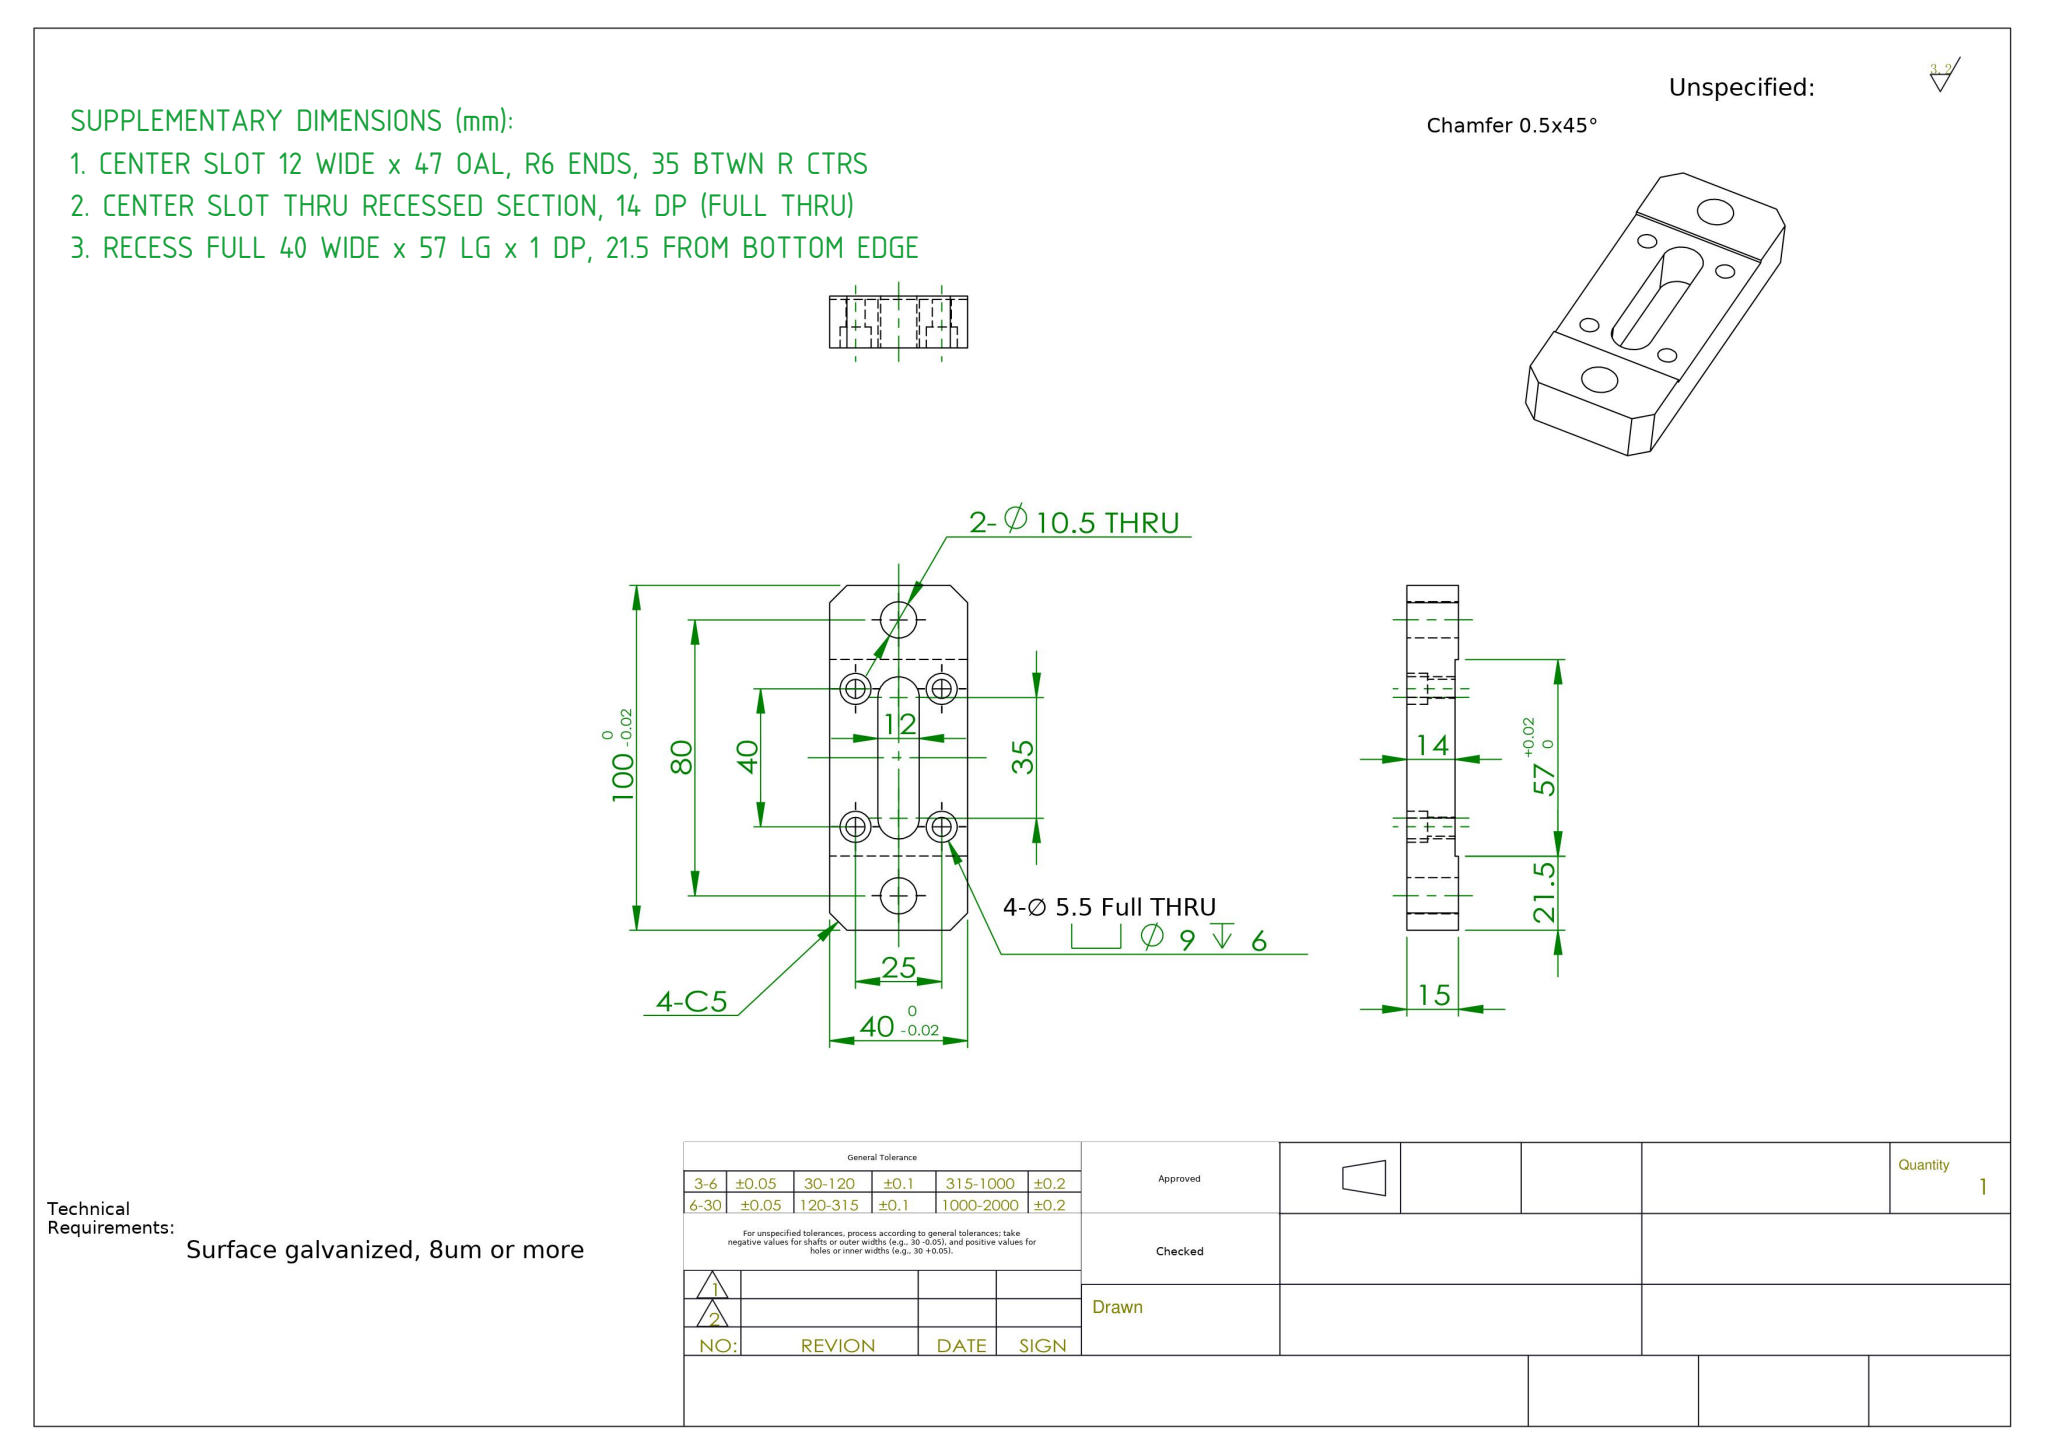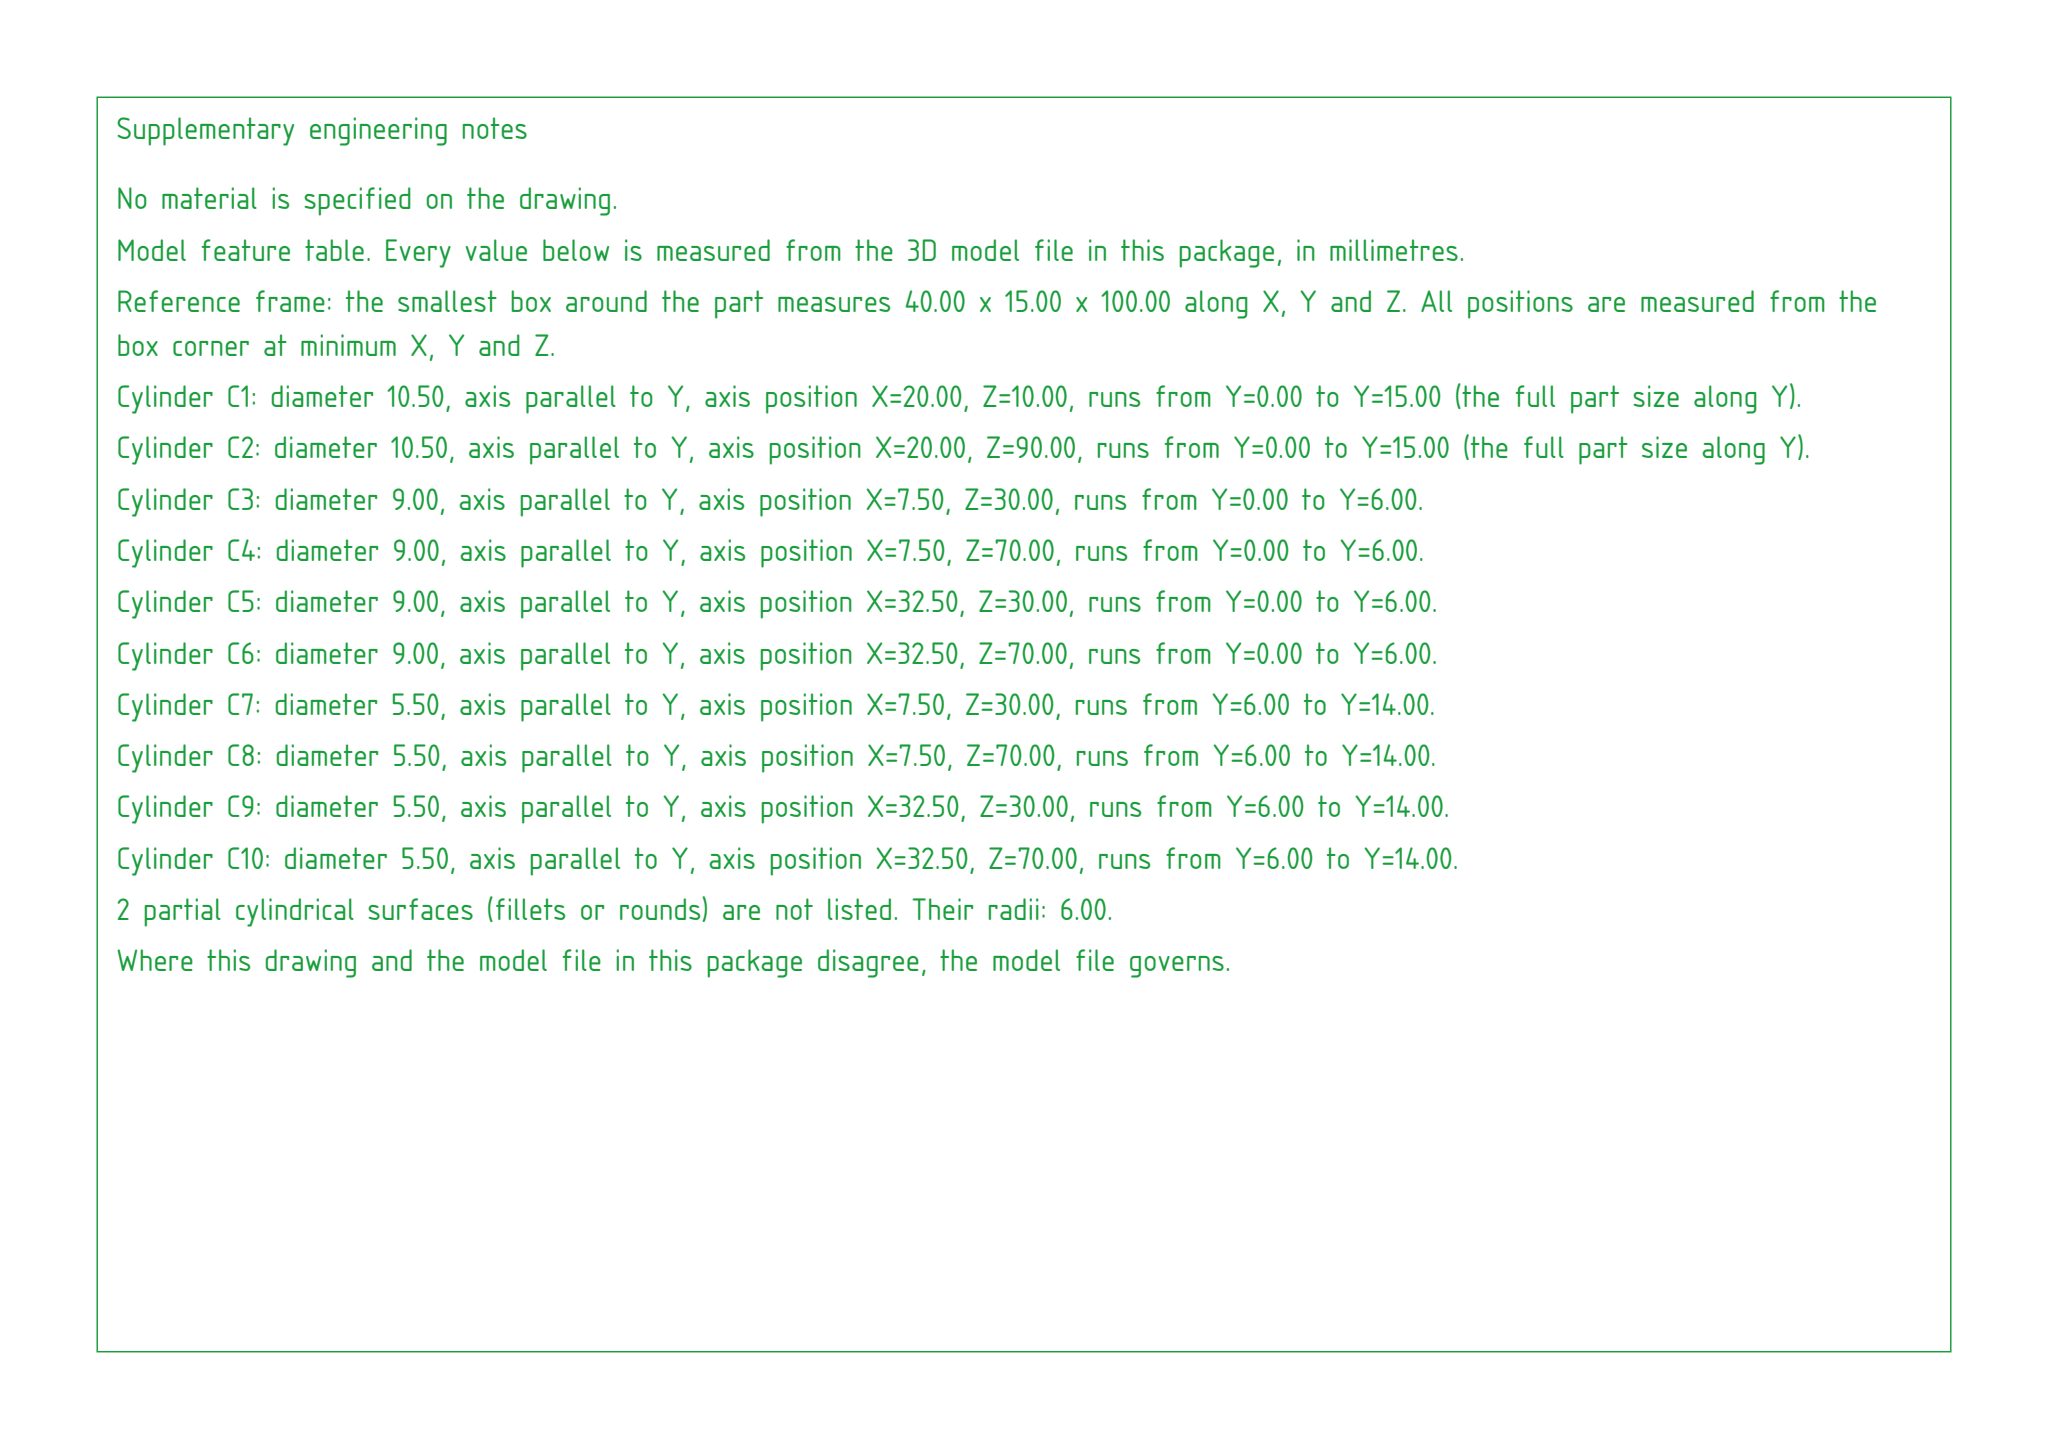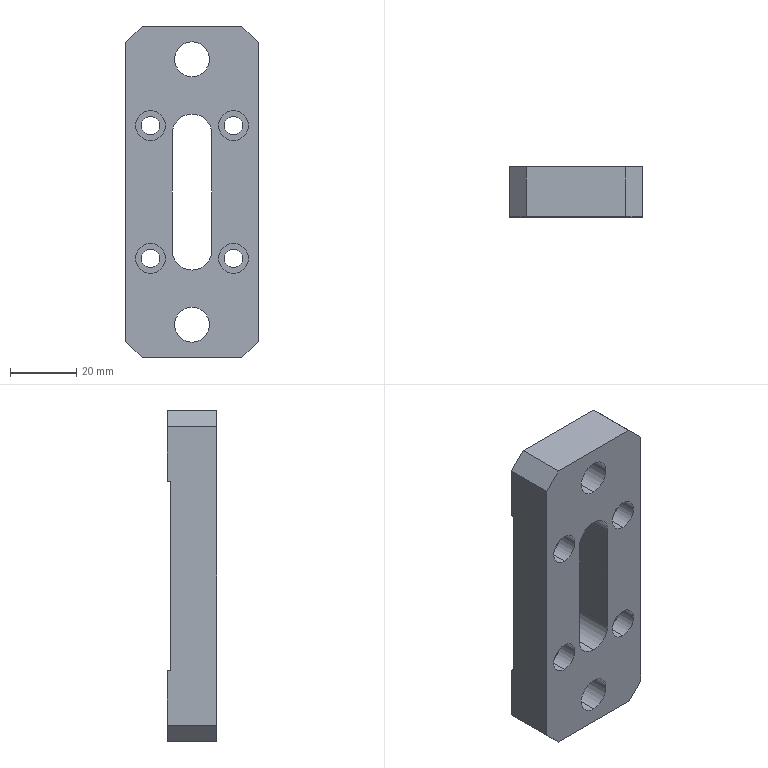Part | SolidWorks | mm | 1 solid | 43 faces | box 40 x 15 x 100 mm | volume 44622 mm3 | cylinder 23 | plane 20 | commonest cylinder face diameters 9 x8 5.5 x8 10.5 x4 12 x3
build123d program:
from build123d import *

# Parameters (mm, degrees)
EXTRUDE1_DEPTH                                  = 20
SKETCH2_R                                       = 5.25
CUT_EXTRUDE1_DEPTH                              = 56.902
M5_HEX_SOCKET_HEAD_CAP_SCREW_CBORE1_D           = 5.5
M5_HEX_SOCKET_HEAD_CAP_SCREW_CBORE1_CBORE_D     = 9
M5_HEX_SOCKET_HEAD_CAP_SCREW_CBORE1_CBORE_DEPTH = 6
MIRROR3_COPY_1_D                                = 5.5
MIRROR3_COPY_1_CBORE_D                          = 9
MIRROR3_COPY_1_CBORE_DEPTH                      = 6
CUT_EXTRUDE2_DEPTH                              = 56.902
CHAMFER1_SIZE                                   = 5


with BuildPart() as part:
    # Sketch1 → Extrude1 (new, symmetric)
    with BuildSketch(Plane(origin=(0, 0, 0), x_dir=(0, 0, -1), z_dir=(1, 0, 0))):
        Polygon((50, 0), (-50, 0), (-50, 15), (-28.5, 15), (-28.5, 14), (28.5, 14), (28.5, 15), (50, 15), align=None)
    extrude(amount=EXTRUDE1_DEPTH, both=True)

    # Sketch2 → Cut-Extrude1 (cut, through all)
    with BuildSketch(Plane(origin=(0, 15, 0), x_dir=(1, 0, 0), z_dir=(0, 1, 0))):
        with Locations(Location((0, -40, 0), (0, 0, 270))):
            Circle(SKETCH2_R)
    cut_extrude1 = extrude(amount=-CUT_EXTRUDE1_DEPTH, mode=Mode.SUBTRACT)

    # Mirror1: Cut-Extrude1 across plane
    add(cut_extrude1.mirror(Plane.XY), mode=Mode.SUBTRACT)

    # M5 Hex Socket Head Cap Screw CBORE1 (through all)
    with Locations(Plane.XZ):
        with Locations((-12.5, -20)):
            m5_hex_socket_head_cap_screw_cbore1 = CounterBoreHole(M5_HEX_SOCKET_HEAD_CAP_SCREW_CBORE1_D / 2, M5_HEX_SOCKET_HEAD_CAP_SCREW_CBORE1_CBORE_D / 2, M5_HEX_SOCKET_HEAD_CAP_SCREW_CBORE1_CBORE_DEPTH)

    # Mirror2: M5 Hex Socket Head Cap Screw CBORE1 across plane
    add(m5_hex_socket_head_cap_screw_cbore1.mirror(Plane(origin=(0, 0, 0), x_dir=(0, 0, 1), z_dir=(1, 0, 0))), mode=Mode.SUBTRACT)

    # Mirror3: M5 Hex Socket Head Cap Screw CBORE1 across plane
    add(m5_hex_socket_head_cap_screw_cbore1.mirror(Plane.XY), mode=Mode.SUBTRACT)

    # Mirror3 copy 1 (through all)
    with Locations(Plane(origin=(0, 0, 0), x_dir=(-1, 0, 0), z_dir=(0, -1, 0))):
        with Locations((-12.5, -20)):
            CounterBoreHole(MIRROR3_COPY_1_D / 2, MIRROR3_COPY_1_CBORE_D / 2, MIRROR3_COPY_1_CBORE_DEPTH)

    # Sketch6 → Cut-Extrude2 (cut, through all)
    with BuildSketch(Plane.XZ):
        with BuildLine():
            Line((-6, -17.5), (-6, 17.5))
            ThreePointArc((-6, 17.5), (0, 23.5), (6, 17.5))
            Line((6, 17.5), (6, -17.5))
            ThreePointArc((6, -17.5), (0, -23.5), (-6, -17.5))
        make_face()
    extrude(amount=-CUT_EXTRUDE2_DEPTH, mode=Mode.SUBTRACT)

    # Chamfer1
    chamfer1_edges = [part.edges().sort_by_distance(p)[0] for p in [
        (20, 7.5, -50),
        (-20, 7.5, 50),
        (20, 7.5, 50),
        (-20, 7.5, -50),
    ]]
    chamfer(chamfer1_edges, length=CHAMFER1_SIZE)


solid = part.part